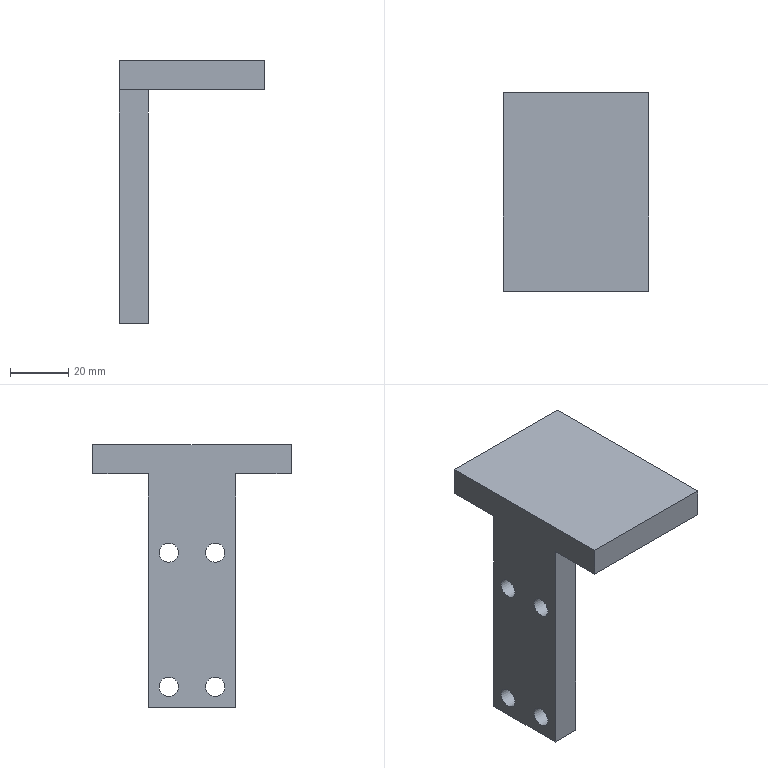Component | NX | GRIPPER_JAW_VERT_PLATE_2 | 1 solid | 18 faces | volume 55749 mm3 | plane 10 | cylinder 6 | cone 2 | commonest cylinder face diameters 6.6 x4 6 x2